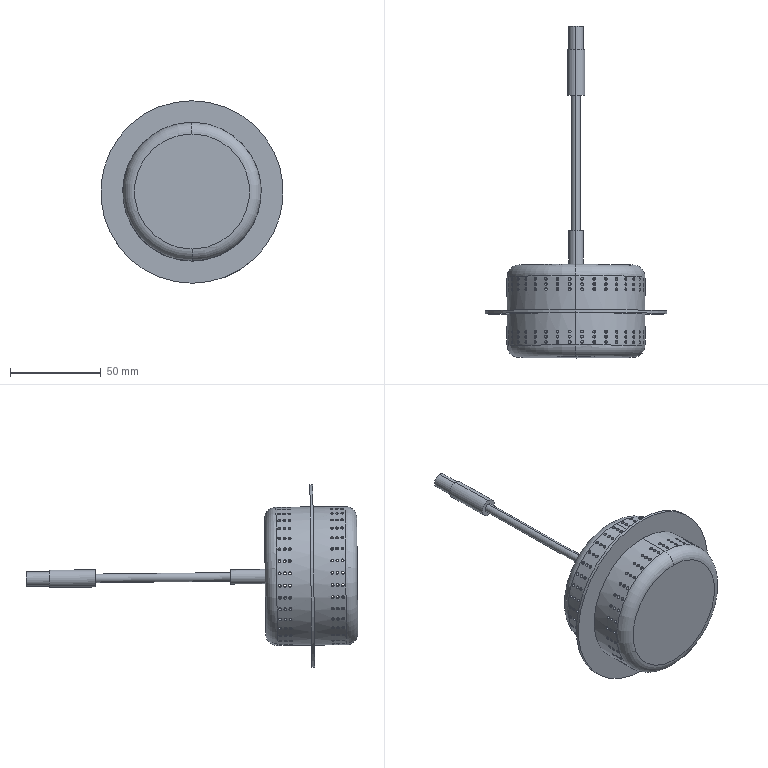Component | NX | CONNECTING_SHAFT | 2 solids | 455 faces | volume 39738 mm3 | cylinder 436 | plane 11 | torus 8 | commonest cylinder face diameters 1.587 x420 76.2 x4 7.938 x2 7.888 x2 4.713 x2 9.476 x2 100.549 x2 73.025 x2